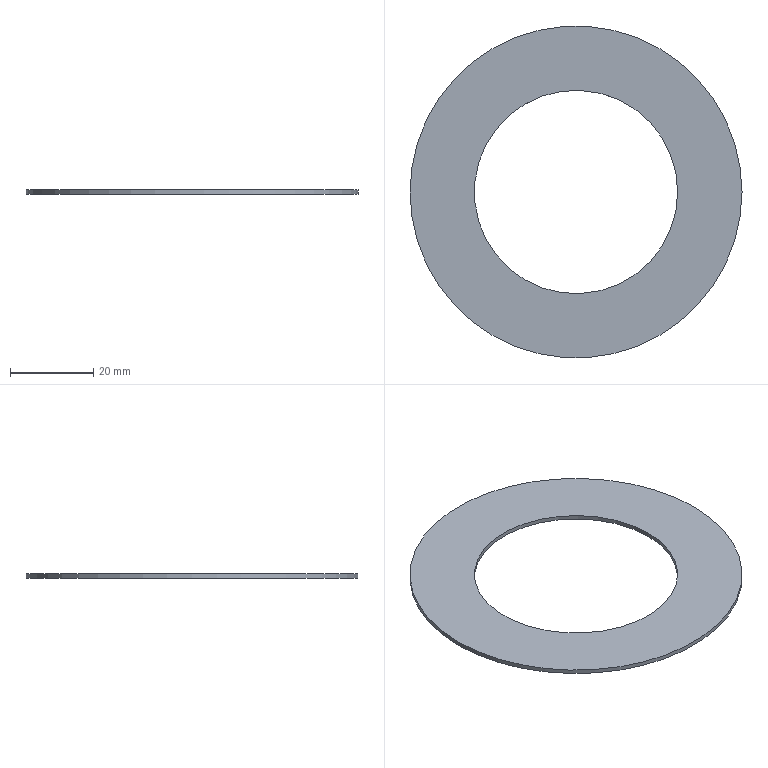Component | NX | CH3404_1-6 | 1 solid | 4 faces | box 80 x 80 x 1 mm | volume 3141 mm3 | cylinder 2 | plane 2 | commonest cylinder face diameters 80 x1 49 x1
STEP:
#1=CARTESIAN_POINT('',(0.,0.,0.));
#2=DIRECTION('',(0.,0.,1.));
#3=DIRECTION('',(1.,0.,0.));
#4=AXIS2_PLACEMENT_3D('',#1,#2,#3);
#5=CARTESIAN_POINT('',(40.,0.,21.));
#6=VERTEX_POINT('',#5);
#7=CARTESIAN_POINT('',(0.,0.,21.));
#8=DIRECTION('',(0.,0.,1.));
#9=DIRECTION('',(1.,0.,0.));
#10=AXIS2_PLACEMENT_3D('',#7,#8,#9);
#11=CIRCLE('',#10,40.);
#12=CARTESIAN_POINT('',(0.,0.,21.));
#13=DIRECTION('',(0.,0.,-1.));
#14=DIRECTION('',(-1.,0.,0.));
#15=AXIS2_PLACEMENT_3D('',#12,#13,#14);
#16=CYLINDRICAL_SURFACE('',#15,40.);
#17=CARTESIAN_POINT('',(9.425,0.));
#18=DIRECTION('',(-1.,0.));
#19=VECTOR('',#18,1.);
#20=LINE('',#17,#19);
#21=(GEOMETRIC_REPRESENTATION_CONTEXT(2)PARAMETRIC_REPRESENTATION_CONTEXT()REPRESENTATION_CONTEXT('',''));
#22=DEFINITIONAL_REPRESENTATION('',(#20),#21);
#23=PCURVE('',#16,#22);
#24=CARTESIAN_POINT('',(0.,0.,21.));
#25=DIRECTION('',(0.,0.,1.));
#26=DIRECTION('',(1.,0.,0.));
#27=AXIS2_PLACEMENT_3D('',#24,#25,#26);
#28=PLANE('',#27);
#29=CARTESIAN_POINT('',(0.,0.));
#30=DIRECTION('',(1.,0.));
#31=AXIS2_PLACEMENT_2D('',#29,#30);
#32=CIRCLE('',#31,40.);
#33=(GEOMETRIC_REPRESENTATION_CONTEXT(2)PARAMETRIC_REPRESENTATION_CONTEXT()REPRESENTATION_CONTEXT('',''));
#34=DEFINITIONAL_REPRESENTATION('',(#32),#33);
#35=PCURVE('',#28,#34);
#36=SURFACE_CURVE('',#11,(#23,#35),.PCURVE_S1.);
#37=EDGE_CURVE('',#6,#6,#36,.T.);
#38=ORIENTED_EDGE('',*,*,#37,.F.);
#39=CARTESIAN_POINT('',(40.,0.,20.));
#40=VERTEX_POINT('',#39);
#41=CARTESIAN_POINT('',(40.,0.,21.));
#42=CARTESIAN_POINT('',(40.,0.,20.));
#43=B_SPLINE_CURVE_WITH_KNOTS('',1,(#41,#42),.UNSPECIFIED.,.F.,.F.,(2,2),(0.,1.),.PIECEWISE_BEZIER_KNOTS.);
#44=CARTESIAN_POINT('',(9.425,0.));
#45=DIRECTION('',(0.,1.));
#46=VECTOR('',#45,1.);
#47=LINE('',#44,#46);
#48=(GEOMETRIC_REPRESENTATION_CONTEXT(2)PARAMETRIC_REPRESENTATION_CONTEXT()REPRESENTATION_CONTEXT('',''));
#49=DEFINITIONAL_REPRESENTATION('',(#47),#48);
#50=PCURVE('',#16,#49);
#51=CARTESIAN_POINT('',(3.142,0.));
#52=DIRECTION('',(0.,1.));
#53=VECTOR('',#52,1.);
#54=LINE('',#51,#53);
#55=(GEOMETRIC_REPRESENTATION_CONTEXT(2)PARAMETRIC_REPRESENTATION_CONTEXT()REPRESENTATION_CONTEXT('',''));
#56=DEFINITIONAL_REPRESENTATION('',(#54),#55);
#57=PCURVE('',#16,#56);
#58=SEAM_CURVE('',#43,(#50,#57),.PCURVE_S1.);
#59=EDGE_CURVE('',#6,#40,#58,.T.);
#60=ORIENTED_EDGE('',*,*,#59,.T.);
#61=CARTESIAN_POINT('',(0.,0.,20.));
#62=DIRECTION('',(0.,0.,1.));
#63=DIRECTION('',(1.,0.,0.));
#64=AXIS2_PLACEMENT_3D('',#61,#62,#63);
#65=CIRCLE('',#64,40.);
#66=CARTESIAN_POINT('',(9.425,1.));
#67=DIRECTION('',(-1.,0.));
#68=VECTOR('',#67,1.);
#69=LINE('',#66,#68);
#70=(GEOMETRIC_REPRESENTATION_CONTEXT(2)PARAMETRIC_REPRESENTATION_CONTEXT()REPRESENTATION_CONTEXT('',''));
#71=DEFINITIONAL_REPRESENTATION('',(#69),#70);
#72=PCURVE('',#16,#71);
#73=CARTESIAN_POINT('',(0.,0.,20.));
#74=DIRECTION('',(0.,0.,1.));
#75=DIRECTION('',(1.,0.,0.));
#76=AXIS2_PLACEMENT_3D('',#73,#74,#75);
#77=PLANE('',#76);
#78=CARTESIAN_POINT('',(0.,0.));
#79=DIRECTION('',(1.,0.));
#80=AXIS2_PLACEMENT_2D('',#78,#79);
#81=CIRCLE('',#80,40.);
#82=(GEOMETRIC_REPRESENTATION_CONTEXT(2)PARAMETRIC_REPRESENTATION_CONTEXT()REPRESENTATION_CONTEXT('',''));
#83=DEFINITIONAL_REPRESENTATION('',(#81),#82);
#84=PCURVE('',#77,#83);
#85=SURFACE_CURVE('',#65,(#72,#84),.PCURVE_S1.);
#86=EDGE_CURVE('',#40,#40,#85,.T.);
#87=ORIENTED_EDGE('',*,*,#86,.T.);
#88=ORIENTED_EDGE('',*,*,#59,.F.);
#89=EDGE_LOOP('',(#38,#60,#87,#88));
#90=FACE_BOUND('',#89,.T.);
#91=ADVANCED_FACE('',(#90),#16,.T.);
#92=CARTESIAN_POINT('',(24.5,0.,21.));
#93=VERTEX_POINT('',#92);
#94=CARTESIAN_POINT('',(0.,0.,21.));
#95=DIRECTION('',(0.,0.,1.));
#96=DIRECTION('',(1.,0.,0.));
#97=AXIS2_PLACEMENT_3D('',#94,#95,#96);
#98=CIRCLE('',#97,24.5);
#99=CARTESIAN_POINT('',(0.,0.,21.));
#100=DIRECTION('',(0.,0.,-1.));
#101=DIRECTION('',(-1.,0.,0.));
#102=AXIS2_PLACEMENT_3D('',#99,#100,#101);
#103=CYLINDRICAL_SURFACE('',#102,24.5);
#104=CARTESIAN_POINT('',(9.425,0.));
#105=DIRECTION('',(-1.,0.));
#106=VECTOR('',#105,1.);
#107=LINE('',#104,#106);
#108=(GEOMETRIC_REPRESENTATION_CONTEXT(2)PARAMETRIC_REPRESENTATION_CONTEXT()REPRESENTATION_CONTEXT('',''));
#109=DEFINITIONAL_REPRESENTATION('',(#107),#108);
#110=PCURVE('',#103,#109);
#111=CARTESIAN_POINT('',(0.,0.));
#112=DIRECTION('',(1.,0.));
#113=AXIS2_PLACEMENT_2D('',#111,#112);
#114=CIRCLE('',#113,24.5);
#115=(GEOMETRIC_REPRESENTATION_CONTEXT(2)PARAMETRIC_REPRESENTATION_CONTEXT()REPRESENTATION_CONTEXT('',''));
#116=DEFINITIONAL_REPRESENTATION('',(#114),#115);
#117=PCURVE('',#28,#116);
#118=SURFACE_CURVE('',#98,(#110,#117),.PCURVE_S1.);
#119=EDGE_CURVE('',#93,#93,#118,.T.);
#120=ORIENTED_EDGE('',*,*,#119,.F.);
#121=CARTESIAN_POINT('',(24.5,0.,20.));
#122=VERTEX_POINT('',#121);
#123=CARTESIAN_POINT('',(24.5,0.,21.));
#124=CARTESIAN_POINT('',(24.5,0.,20.));
#125=B_SPLINE_CURVE_WITH_KNOTS('',1,(#123,#124),.UNSPECIFIED.,.F.,.F.,(2,2),(0.,1.),.PIECEWISE_BEZIER_KNOTS.);
#126=CARTESIAN_POINT('',(9.425,0.));
#127=DIRECTION('',(0.,1.));
#128=VECTOR('',#127,1.);
#129=LINE('',#126,#128);
#130=(GEOMETRIC_REPRESENTATION_CONTEXT(2)PARAMETRIC_REPRESENTATION_CONTEXT()REPRESENTATION_CONTEXT('',''));
#131=DEFINITIONAL_REPRESENTATION('',(#129),#130);
#132=PCURVE('',#103,#131);
#133=CARTESIAN_POINT('',(3.142,0.));
#134=DIRECTION('',(0.,1.));
#135=VECTOR('',#134,1.);
#136=LINE('',#133,#135);
#137=(GEOMETRIC_REPRESENTATION_CONTEXT(2)PARAMETRIC_REPRESENTATION_CONTEXT()REPRESENTATION_CONTEXT('',''));
#138=DEFINITIONAL_REPRESENTATION('',(#136),#137);
#139=PCURVE('',#103,#138);
#140=SEAM_CURVE('',#125,(#132,#139),.PCURVE_S1.);
#141=EDGE_CURVE('',#93,#122,#140,.T.);
#142=ORIENTED_EDGE('',*,*,#141,.T.);
#143=CARTESIAN_POINT('',(0.,0.,20.));
#144=DIRECTION('',(0.,0.,1.));
#145=DIRECTION('',(1.,0.,0.));
#146=AXIS2_PLACEMENT_3D('',#143,#144,#145);
#147=CIRCLE('',#146,24.5);
#148=CARTESIAN_POINT('',(9.425,1.));
#149=DIRECTION('',(-1.,0.));
#150=VECTOR('',#149,1.);
#151=LINE('',#148,#150);
#152=(GEOMETRIC_REPRESENTATION_CONTEXT(2)PARAMETRIC_REPRESENTATION_CONTEXT()REPRESENTATION_CONTEXT('',''));
#153=DEFINITIONAL_REPRESENTATION('',(#151),#152);
#154=PCURVE('',#103,#153);
#155=CARTESIAN_POINT('',(0.,0.));
#156=DIRECTION('',(1.,0.));
#157=AXIS2_PLACEMENT_2D('',#155,#156);
#158=CIRCLE('',#157,24.5);
#159=(GEOMETRIC_REPRESENTATION_CONTEXT(2)PARAMETRIC_REPRESENTATION_CONTEXT()REPRESENTATION_CONTEXT('',''));
#160=DEFINITIONAL_REPRESENTATION('',(#158),#159);
#161=PCURVE('',#77,#160);
#162=SURFACE_CURVE('',#147,(#154,#161),.PCURVE_S1.);
#163=EDGE_CURVE('',#122,#122,#162,.T.);
#164=ORIENTED_EDGE('',*,*,#163,.T.);
#165=ORIENTED_EDGE('',*,*,#141,.F.);
#166=EDGE_LOOP('',(#120,#142,#164,#165));
#167=FACE_BOUND('',#166,.F.);
#168=ADVANCED_FACE('',(#167),#103,.F.);
#169=ORIENTED_EDGE('',*,*,#37,.T.);
#170=EDGE_LOOP('',(#169));
#171=FACE_BOUND('',#170,.T.);
#172=ORIENTED_EDGE('',*,*,#119,.F.);
#173=EDGE_LOOP('',(#172));
#174=FACE_BOUND('',#173,.T.);
#175=ADVANCED_FACE('',(#171,#174),#28,.T.);
#176=ORIENTED_EDGE('',*,*,#86,.F.);
#177=EDGE_LOOP('',(#176));
#178=FACE_BOUND('',#177,.T.);
#179=ORIENTED_EDGE('',*,*,#163,.T.);
#180=EDGE_LOOP('',(#179));
#181=FACE_BOUND('',#180,.T.);
#182=ADVANCED_FACE('',(#178,#181),#77,.F.);
#183=CLOSED_SHELL('',(#91,#168,#175,#182));
#184=MANIFOLD_SOLID_BREP('',#183);
#185=(LENGTH_UNIT()NAMED_UNIT(*)SI_UNIT(.MILLI.,.METRE.));
#186=UNCERTAINTY_MEASURE_WITH_UNIT(LENGTH_MEASURE(0.00001),#185,'','');
#187=(NAMED_UNIT(*)PLANE_ANGLE_UNIT()SI_UNIT($,.RADIAN.));
#188=(NAMED_UNIT(*)SI_UNIT($,.STERADIAN.)SOLID_ANGLE_UNIT());
#189=(GEOMETRIC_REPRESENTATION_CONTEXT(3)GLOBAL_UNCERTAINTY_ASSIGNED_CONTEXT((#186))GLOBAL_UNIT_ASSIGNED_CONTEXT((#185,#187,#188))REPRESENTATION_CONTEXT('',''));
#190=ADVANCED_BREP_SHAPE_REPRESENTATION('',(#4,#184),#189);